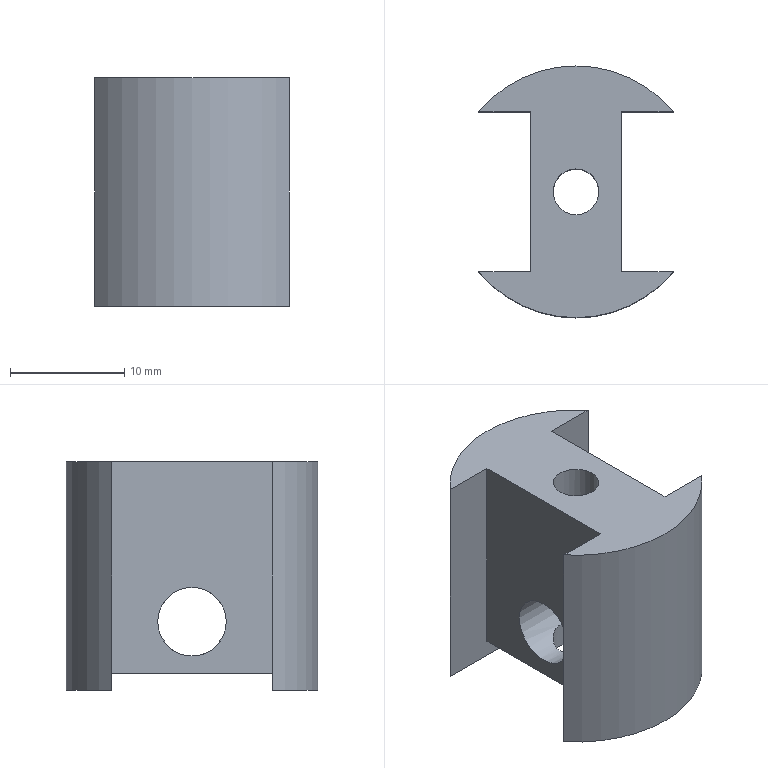Component | NX | 18C__27 | 1 solid | 13 faces | volume 3573 mm3 | plane 8 | cylinder 5 | commonest cylinder face diameters 4 x2 22 x2 6 x1